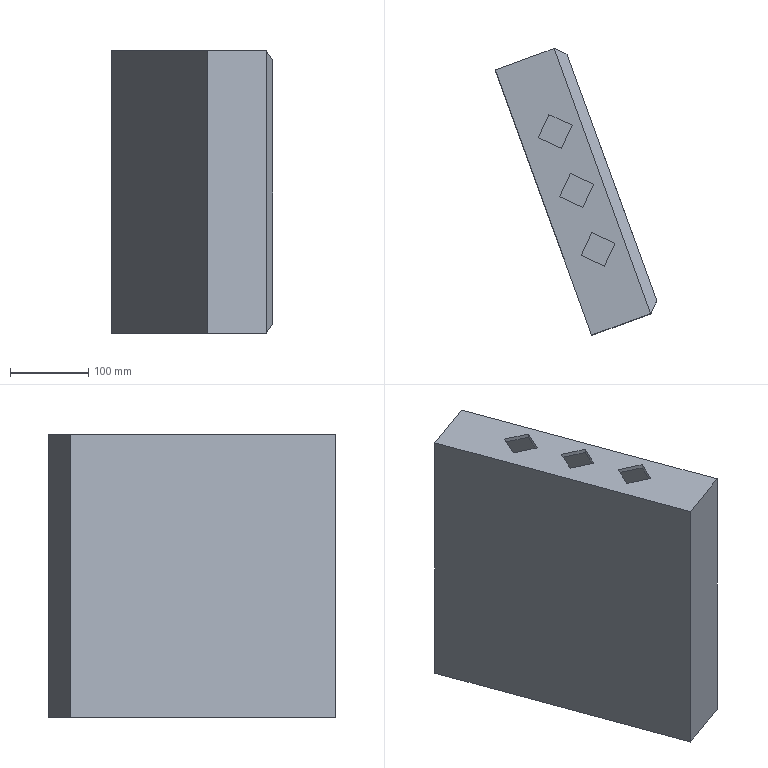Component | NX | AIR_OUTLET_DEVICE_2 | 1 solid | 56 faces | volume 1745357 mm3 | plane 48 | cylinder 8 | commonest cylinder face diameters 200 x8